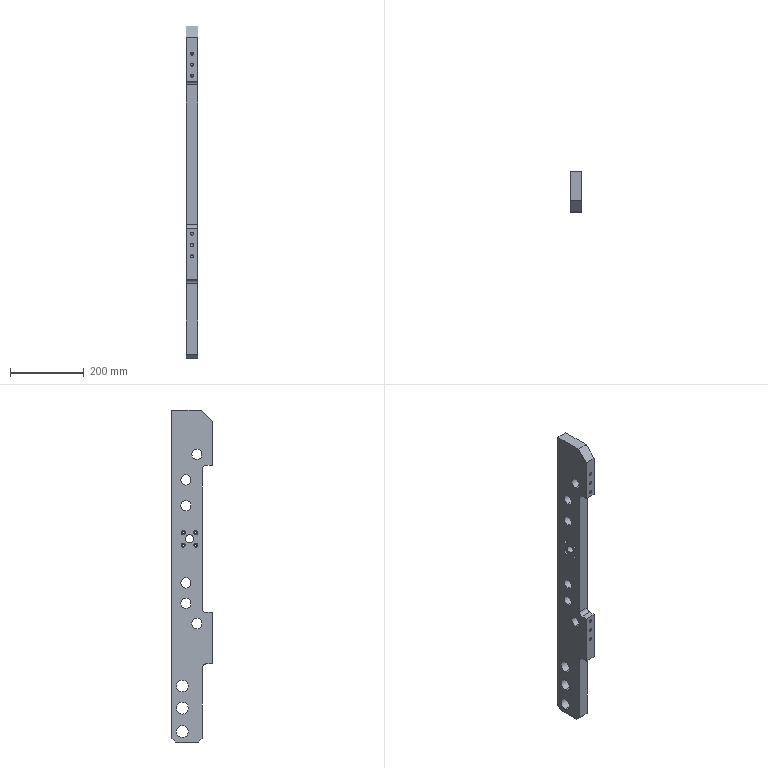Component | SolidWorks | EE8-211-_+-_T_w_O(_k)-1 | 1 solid | 107 faces | box 30 x 109.5 x 902 mm | volume 2222112 mm3 | cylinder 65 | plane 22 | cone 20 | commonest cylinder face diameters 28 x12 8.5 x12 11 x8 6.6 x8 10.2 x8 45 x6 32 x6 20 x3
build123d program:
from build123d import *

# Parameters (mm, degrees)
SKETCH1_W                                            = 902
SKETCH1_H                                            = 109.5
BOSS_EXTRUDE1_DEPTH                                  = 15
SKETCH2_W                                            = 400
SKETCH2_H                                            = 27
SKETCH2_W_2                                          = 212
CUT_EXTRUDE1_DEPTH                                   = 564.555
FILLET1_10_R                                         = 10
CHAMFER1_30_SIZE                                     = 30
CHAMFER2_10_SIZE                                     = 10
M12X1_75_TAPPED_HOLE_DRILL1_D                        = 10.2
M12X1_75_TAPPED_HOLE_DRILL1_DEPTH                    = 18
M12X1_75_TAPPED_HOLE_DRILL1_TIP                      = 3.064
M10X1_5_TAPPED_HOLE_DRILL1_D                         = 8.5
M10X1_5_TAPPED_HOLE_DRILL1_DEPTH                     = 15
M10X1_5_TAPPED_HOLE_DRILL1_TIP                       = 2.554
F_28_0_28_DIAMETER_HOLE1_D                           = 28
F_22_0_22_DIAMETER_HOLE1_D                           = 22
M30X3_5_TAPPED_HOLE_DRILL1_D                         = 32
COUNTERBORE_FOR_M6_SOCKET_HEAD_CAP_SCREW_D           = 6.6
COUNTERBORE_FOR_M6_SOCKET_HEAD_CAP_SCREW_CBORE_D     = 11
COUNTERBORE_FOR_M6_SOCKET_HEAD_CAP_SCREW_CBORE_DEPTH = 6
SKETCH17_R                                           = 22.5
CUT_EXTRUDE2_DEPTH                                   = 8


with BuildPart() as part:
    # Sketch1 → Boss-Extrude1 (new, symmetric)
    with BuildSketch(Plane.XY):
        with Locations((101, 54.75)):
            Rectangle(SKETCH1_W, SKETCH1_H)
    extrude(amount=BOSS_EXTRUDE1_DEPTH, both=True)

    # Sketch2 → Cut-Extrude1 (cut, through all)
    with BuildSketch(Plane.XY.offset(15)):
        with Locations((0, 13.5)):
            Rectangle(SKETCH2_W, SKETCH2_H)
        with Locations((446, 13.5)):
            Rectangle(SKETCH2_W_2, SKETCH2_H)
    extrude(amount=-CUT_EXTRUDE1_DEPTH, mode=Mode.SUBTRACT)

    # Fillet1-10
    fillet1_10_edges = [part.edges().sort_by_distance(p)[0] for p in [
        (-200, 27, 0),
        (200, 27, 0),
        (340, 27, 0),
    ]]
    fillet(fillet1_10_edges, radius=FILLET1_10_R)

    # Chamfer1-30
    chamfer1_30_edges = [part.edges().sort_by_distance(p)[0] for p in [
        (-350, 0, 0),
    ]]
    chamfer(chamfer1_30_edges, length=CHAMFER1_30_SIZE)

    # Chamfer2-10
    chamfer2_10_edges = [part.edges().sort_by_distance(p)[0] for p in [
        (552, 27, 0),
        (552, 109.5, 0),
    ]]
    chamfer(chamfer2_10_edges, length=CHAMFER2_10_SIZE)

    # M12x1.75 Tapped Hole Drill1
    with Locations(Plane(origin=(0, 109.5, 0), x_dir=(1, 0, 0), z_dir=(0, 1, 0))):
        with Locations((-330, 0), (-298, 0), (210, 0), (235, 0)):
            Hole(M12X1_75_TAPPED_HOLE_DRILL1_D / 2, depth=M12X1_75_TAPPED_HOLE_DRILL1_DEPTH)
            with Locations((0, 0, -(M12X1_75_TAPPED_HOLE_DRILL1_DEPTH + M12X1_75_TAPPED_HOLE_DRILL1_TIP / 2))):  # 118° drill point
                Cone(0, M12X1_75_TAPPED_HOLE_DRILL1_D / 2, M12X1_75_TAPPED_HOLE_DRILL1_TIP, mode=Mode.SUBTRACT)

    # M10x1.5 Tapped Hole Drill1
    with Locations(Plane(origin=(0, 0, 0), x_dir=(-1, 0, 0), z_dir=(0, -1, 0))):
        with Locations((215, 0), (245, 0), (275, 0), (-275, 0), (-245, 0), (-215, 0)):
            Hole(M10X1_5_TAPPED_HOLE_DRILL1_D / 2, depth=M10X1_5_TAPPED_HOLE_DRILL1_DEPTH)
            with Locations((0, 0, -(M10X1_5_TAPPED_HOLE_DRILL1_DEPTH + M10X1_5_TAPPED_HOLE_DRILL1_TIP / 2))):  # 118° drill point
                Cone(0, M10X1_5_TAPPED_HOLE_DRILL1_D / 2, M10X1_5_TAPPED_HOLE_DRILL1_TIP, mode=Mode.SUBTRACT)

    # 28.0 _28_ Diameter Hole1 (through all)
    with Locations(Plane.XY.offset(15)):
        with Locations((-230, 41.5), (-160, 71.5), (-90, 71.5), (120, 71.5), (175, 71.5), (230, 41.5)):
            Hole(F_28_0_28_DIAMETER_HOLE1_D / 2)

    # 22.0 _22_ Diameter Hole1 (through all)
    with Locations(Plane.XY.offset(15)):
        with Locations((0, 61.5)):
            Hole(F_22_0_22_DIAMETER_HOLE1_D / 2)

    # M30x3.5 Tapped Hole Drill1 (through all)
    with Locations(Plane.XY.offset(15)):
        with Locations((400, 81), (460, 81), (524, 81)):
            Hole(M30X3_5_TAPPED_HOLE_DRILL1_D / 2)

    # Counterbore for M6 Socket Head Cap Screw (through all)
    with Locations(Plane(origin=(0, 0, -15), x_dir=(-1, 0, 0), z_dir=(0, 0, -1))):
        with Locations((-17, 78.5), (-17, 44.5), (17, 44.5), (17, 78.5)):
            CounterBoreHole(COUNTERBORE_FOR_M6_SOCKET_HEAD_CAP_SCREW_D / 2, COUNTERBORE_FOR_M6_SOCKET_HEAD_CAP_SCREW_CBORE_D / 2, COUNTERBORE_FOR_M6_SOCKET_HEAD_CAP_SCREW_CBORE_DEPTH)

    # Sketch17 → Cut-Extrude2 (cut)
    with BuildSketch(Plane.XY.offset(15)):
        with Locations((400, 81)):
            Circle(SKETCH17_R)
        with Locations((460, 81)):
            Circle(SKETCH17_R)
        with Locations((524, 81)):
            Circle(SKETCH17_R)
    extrude(amount=-CUT_EXTRUDE2_DEPTH, mode=Mode.SUBTRACT)


solid = part.part

# Placed as in the assembly
solid = solid.moved(Location((0, 0, 0), (0, 90, 0)))